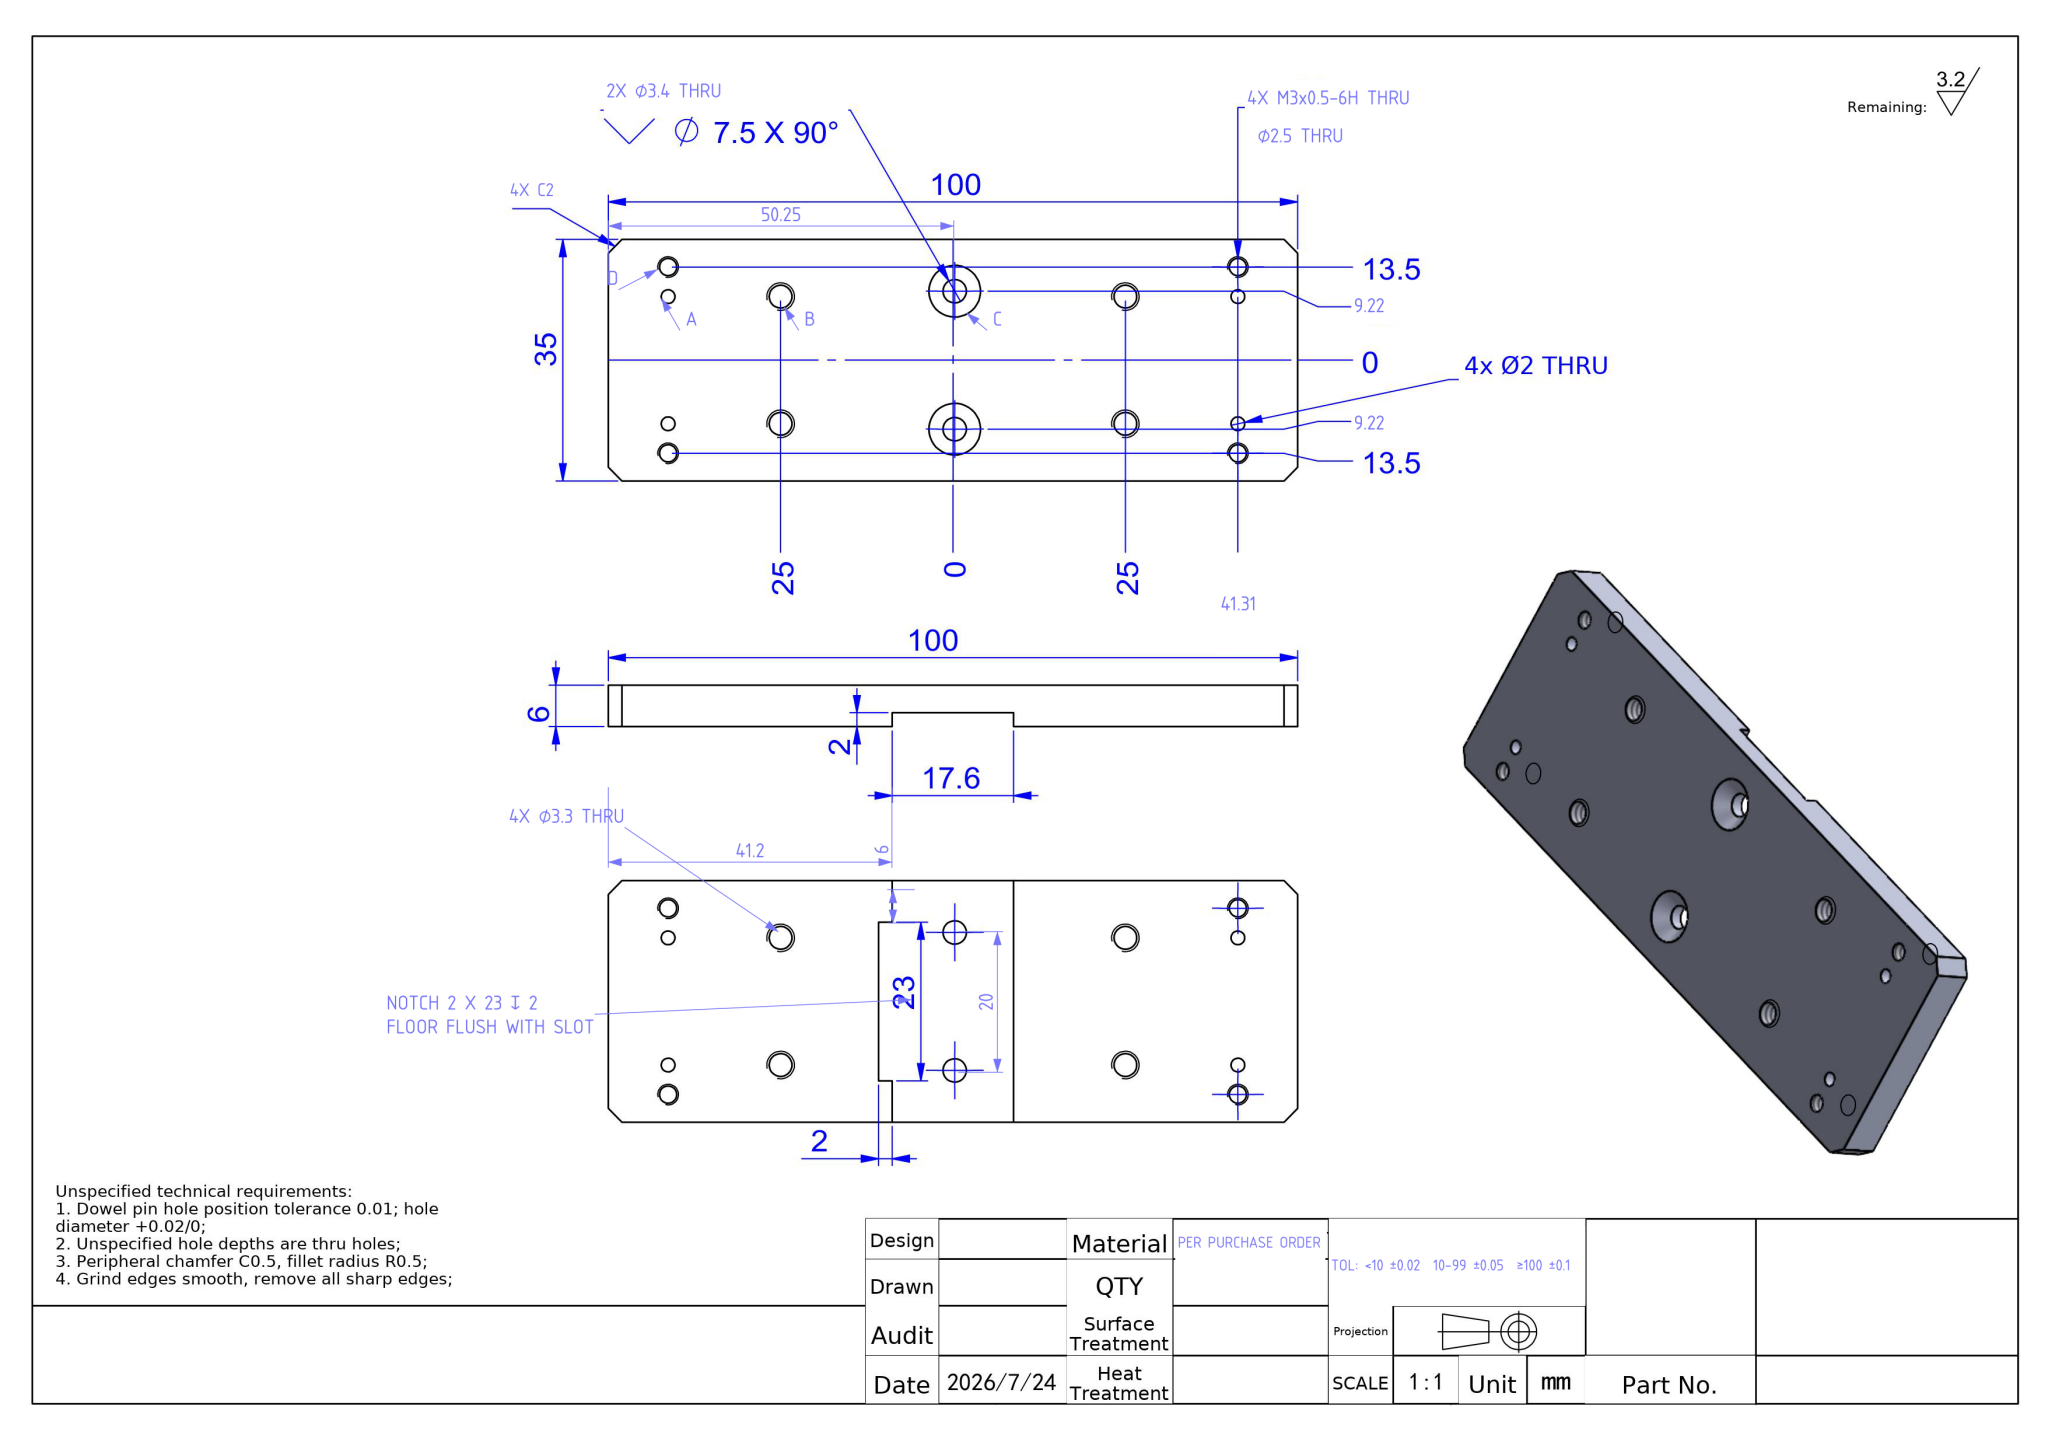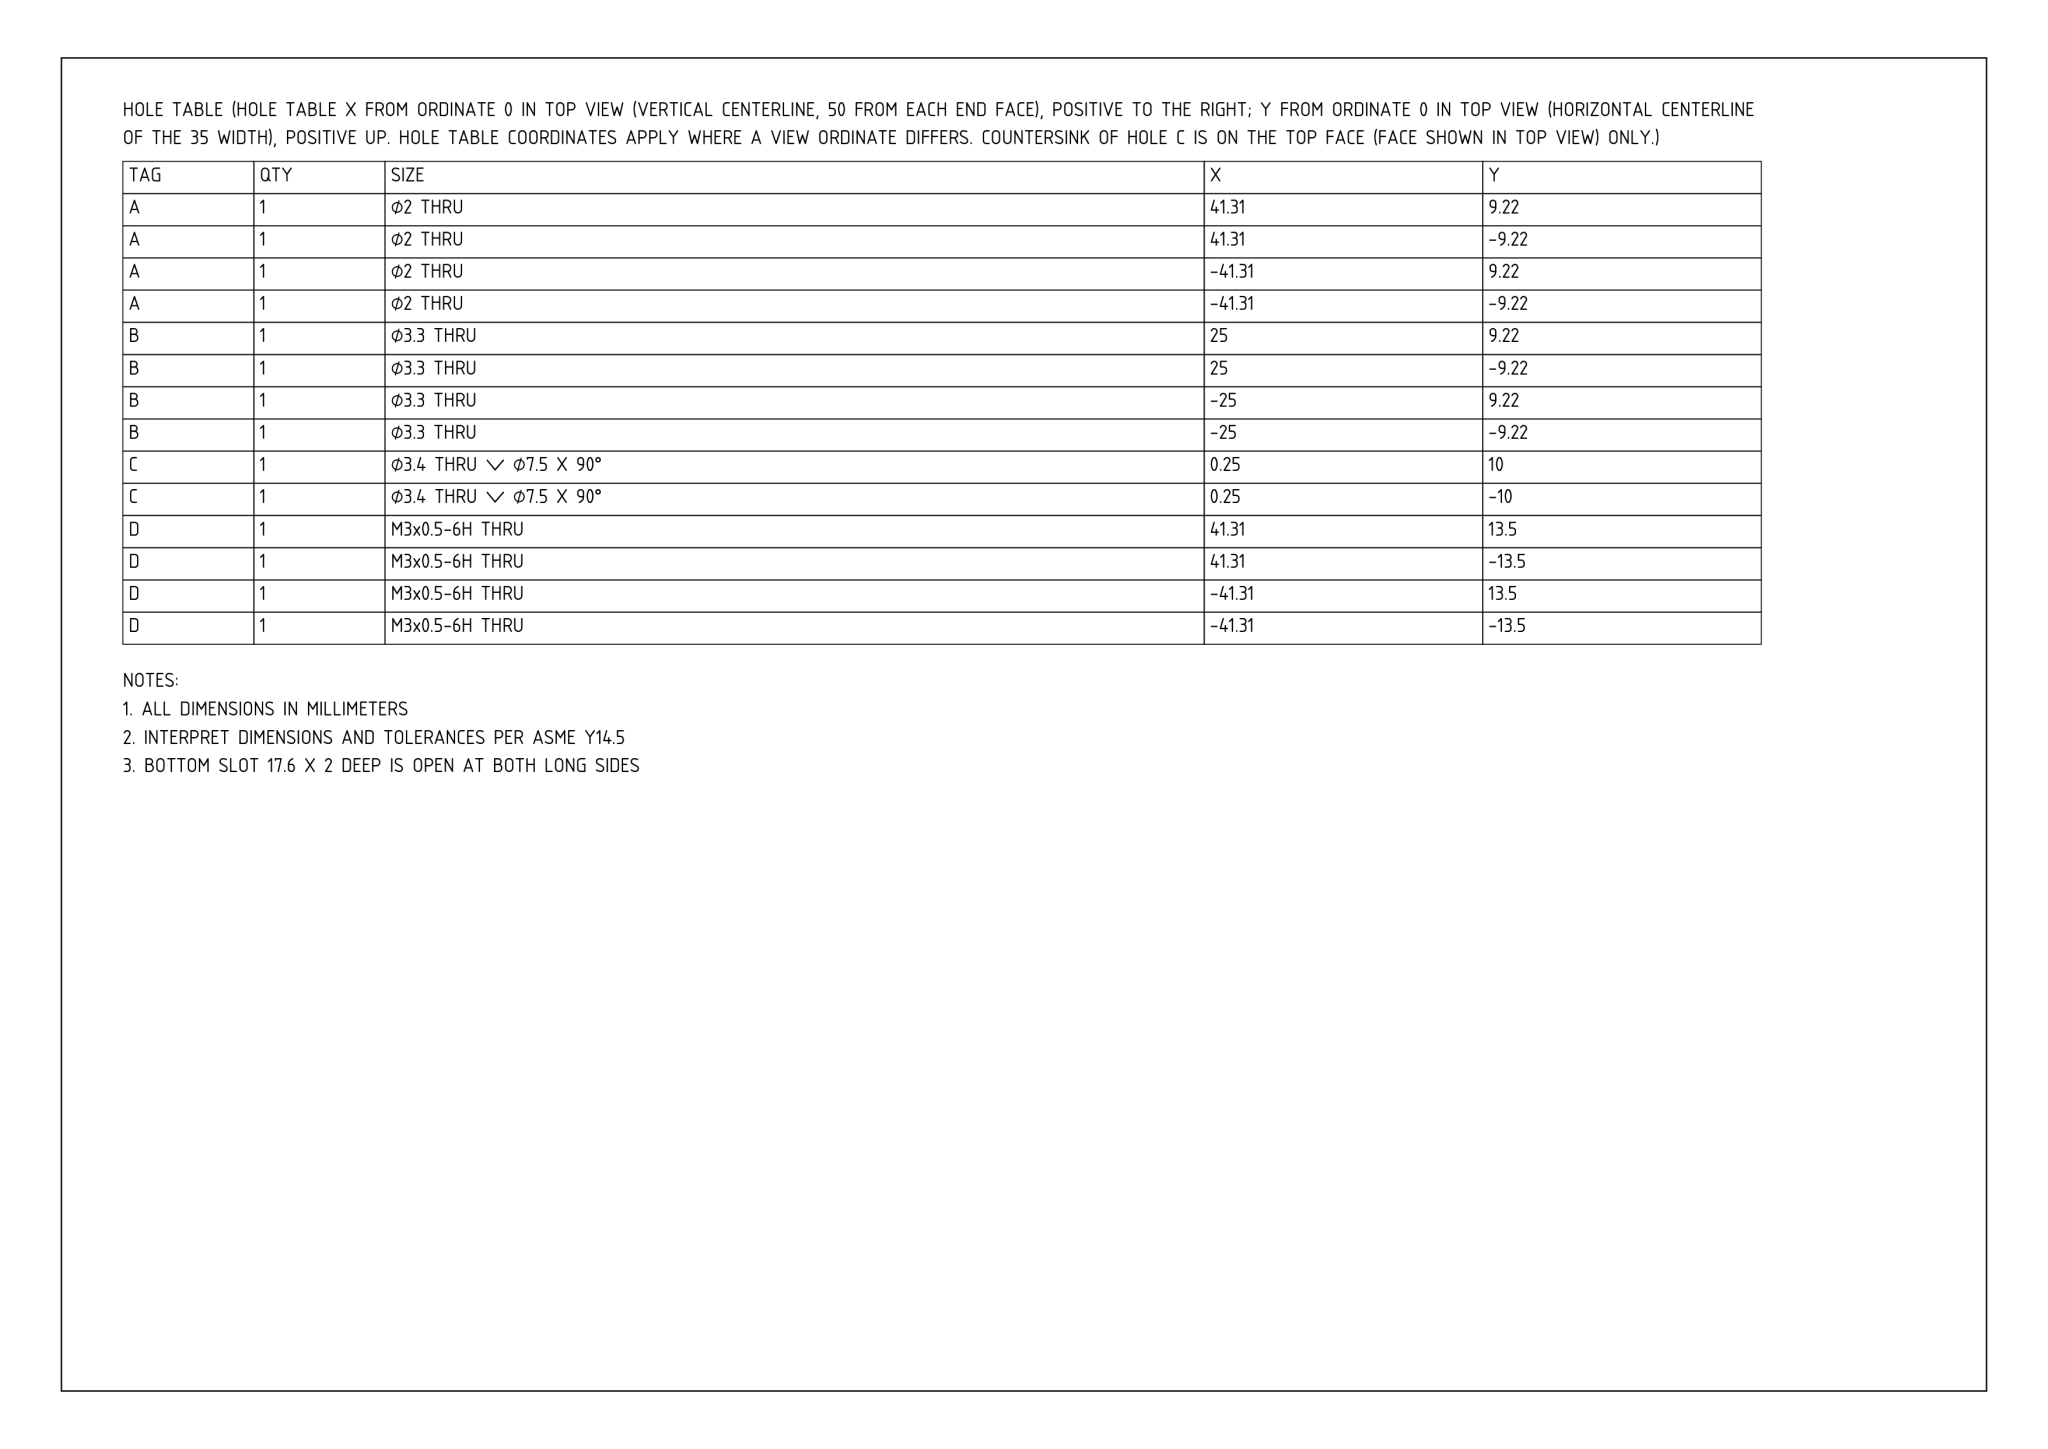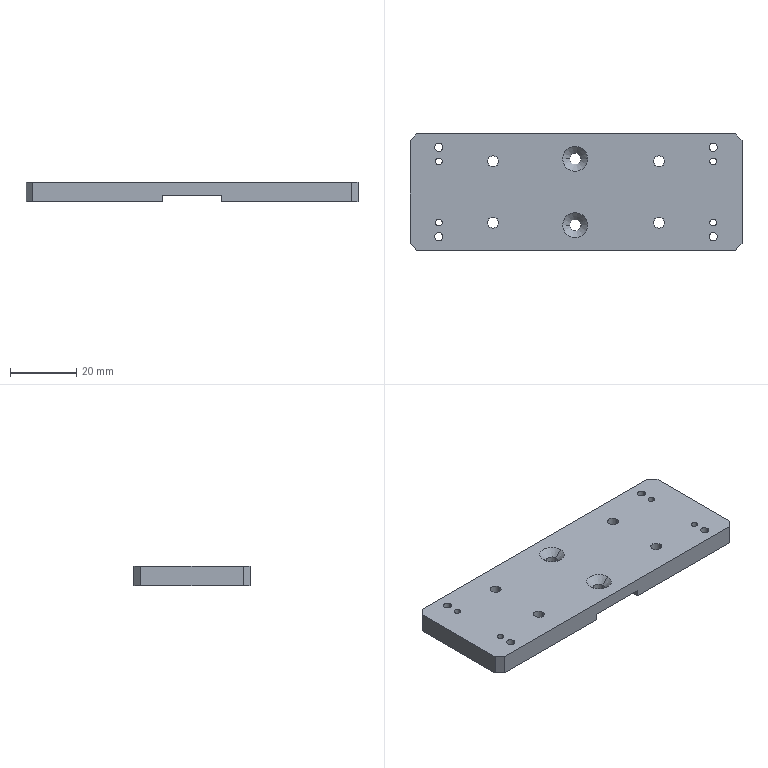Part | NX | mm | 1 solid | 50 faces | box 100 x 35 x 6 mm | volume 19094 mm3 | cylinder 28 | plane 18 | cone 4 | commonest cylinder face diameters 2 x8 2.5 x8 3.3 x8 3.4 x4